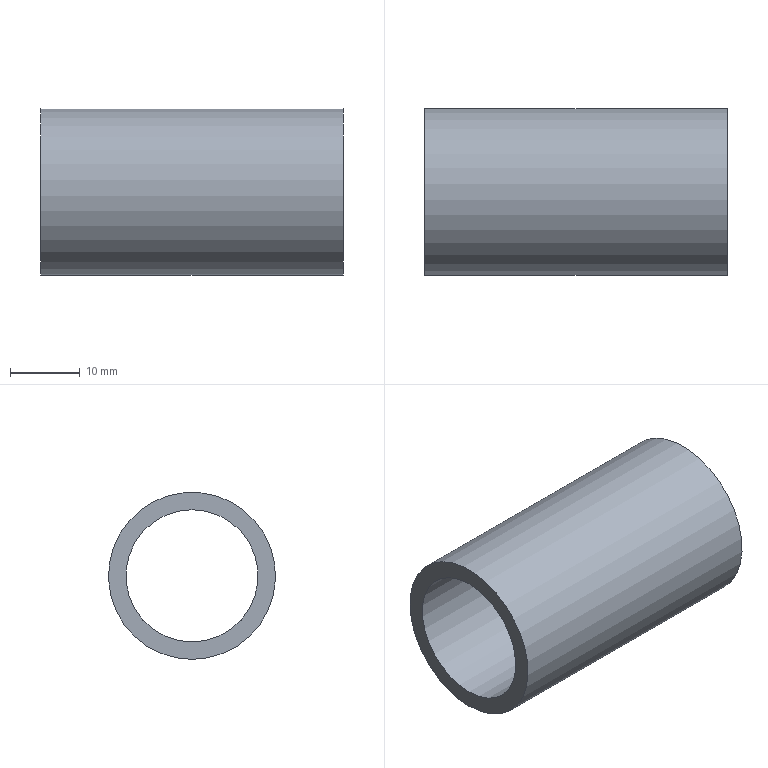Component | NX | LONG_BUSHING | 1 solid | 4 faces | box 43.5 x 24 x 24 mm | volume 7345 mm3 | cylinder 2 | plane 2 | commonest cylinder face diameters 24 x1 19 x1
STEP:
#1=CARTESIAN_POINT('',(0.,0.,0.));
#2=DIRECTION('',(0.,0.,1.));
#3=DIRECTION('',(1.,0.,0.));
#4=AXIS2_PLACEMENT_3D('',#1,#2,#3);
#5=CARTESIAN_POINT('',(-19.,0.,111.));
#6=VERTEX_POINT('',#5);
#7=CARTESIAN_POINT('',(-19.,0.,123.));
#8=DIRECTION('',(-1.,0.,0.));
#9=DIRECTION('',(0.,0.,-1.));
#10=AXIS2_PLACEMENT_3D('',#7,#8,#9);
#11=CIRCLE('',#10,12.);
#12=CARTESIAN_POINT('',(-19.,0.,123.));
#13=DIRECTION('',(-1.,0.,0.));
#14=DIRECTION('',(0.,0.,1.));
#15=AXIS2_PLACEMENT_3D('',#12,#13,#14);
#16=CYLINDRICAL_SURFACE('',#15,12.);
#17=CARTESIAN_POINT('',(3.142,0.));
#18=DIRECTION('',(1.,0.));
#19=VECTOR('',#18,1.);
#20=LINE('',#17,#19);
#21=(GEOMETRIC_REPRESENTATION_CONTEXT(2)PARAMETRIC_REPRESENTATION_CONTEXT()REPRESENTATION_CONTEXT('',''));
#22=DEFINITIONAL_REPRESENTATION('',(#20),#21);
#23=PCURVE('',#16,#22);
#24=CARTESIAN_POINT('',(-19.,0.,123.));
#25=DIRECTION('',(-1.,0.,0.));
#26=DIRECTION('',(0.,0.,1.));
#27=AXIS2_PLACEMENT_3D('',#24,#25,#26);
#28=PLANE('',#27);
#29=CARTESIAN_POINT('',(0.,0.));
#30=DIRECTION('',(-1.,0.));
#31=AXIS2_PLACEMENT_2D('',#29,#30);
#32=CIRCLE('',#31,12.);
#33=(GEOMETRIC_REPRESENTATION_CONTEXT(2)PARAMETRIC_REPRESENTATION_CONTEXT()REPRESENTATION_CONTEXT('',''));
#34=DEFINITIONAL_REPRESENTATION('',(#32),#33);
#35=PCURVE('',#28,#34);
#36=SURFACE_CURVE('',#11,(#23,#35),.PCURVE_S1.);
#37=EDGE_CURVE('',#6,#6,#36,.T.);
#38=ORIENTED_EDGE('',*,*,#37,.T.);
#39=CARTESIAN_POINT('',(-62.5,0.,111.));
#40=VERTEX_POINT('',#39);
#41=CARTESIAN_POINT('',(-19.,0.,111.));
#42=CARTESIAN_POINT('',(-62.5,0.,111.));
#43=B_SPLINE_CURVE_WITH_KNOTS('',1,(#41,#42),.UNSPECIFIED.,.F.,.F.,(2,2),(0.,43.5),.PIECEWISE_BEZIER_KNOTS.);
#44=CARTESIAN_POINT('',(9.425,0.));
#45=DIRECTION('',(0.,1.));
#46=VECTOR('',#45,1.);
#47=LINE('',#44,#46);
#48=(GEOMETRIC_REPRESENTATION_CONTEXT(2)PARAMETRIC_REPRESENTATION_CONTEXT()REPRESENTATION_CONTEXT('',''));
#49=DEFINITIONAL_REPRESENTATION('',(#47),#48);
#50=PCURVE('',#16,#49);
#51=CARTESIAN_POINT('',(3.142,0.));
#52=DIRECTION('',(0.,1.));
#53=VECTOR('',#52,1.);
#54=LINE('',#51,#53);
#55=(GEOMETRIC_REPRESENTATION_CONTEXT(2)PARAMETRIC_REPRESENTATION_CONTEXT()REPRESENTATION_CONTEXT('',''));
#56=DEFINITIONAL_REPRESENTATION('',(#54),#55);
#57=PCURVE('',#16,#56);
#58=SEAM_CURVE('',#43,(#50,#57),.PCURVE_S1.);
#59=EDGE_CURVE('',#6,#40,#58,.T.);
#60=ORIENTED_EDGE('',*,*,#59,.T.);
#61=CARTESIAN_POINT('',(-62.5,0.,123.));
#62=DIRECTION('',(-1.,0.,0.));
#63=DIRECTION('',(0.,0.,-1.));
#64=AXIS2_PLACEMENT_3D('',#61,#62,#63);
#65=CIRCLE('',#64,12.);
#66=CARTESIAN_POINT('',(3.142,43.5));
#67=DIRECTION('',(1.,0.));
#68=VECTOR('',#67,1.);
#69=LINE('',#66,#68);
#70=(GEOMETRIC_REPRESENTATION_CONTEXT(2)PARAMETRIC_REPRESENTATION_CONTEXT()REPRESENTATION_CONTEXT('',''));
#71=DEFINITIONAL_REPRESENTATION('',(#69),#70);
#72=PCURVE('',#16,#71);
#73=CARTESIAN_POINT('',(-62.5,0.,123.));
#74=DIRECTION('',(-1.,0.,0.));
#75=DIRECTION('',(0.,0.,1.));
#76=AXIS2_PLACEMENT_3D('',#73,#74,#75);
#77=PLANE('',#76);
#78=CARTESIAN_POINT('',(0.,0.));
#79=DIRECTION('',(-1.,0.));
#80=AXIS2_PLACEMENT_2D('',#78,#79);
#81=CIRCLE('',#80,12.);
#82=(GEOMETRIC_REPRESENTATION_CONTEXT(2)PARAMETRIC_REPRESENTATION_CONTEXT()REPRESENTATION_CONTEXT('',''));
#83=DEFINITIONAL_REPRESENTATION('',(#81),#82);
#84=PCURVE('',#77,#83);
#85=SURFACE_CURVE('',#65,(#72,#84),.PCURVE_S1.);
#86=EDGE_CURVE('',#40,#40,#85,.T.);
#87=ORIENTED_EDGE('',*,*,#86,.F.);
#88=ORIENTED_EDGE('',*,*,#59,.F.);
#89=EDGE_LOOP('',(#38,#60,#87,#88));
#90=FACE_BOUND('',#89,.T.);
#91=ADVANCED_FACE('',(#90),#16,.T.);
#92=CARTESIAN_POINT('',(-19.,0.,113.5));
#93=VERTEX_POINT('',#92);
#94=CARTESIAN_POINT('',(-19.,0.,123.));
#95=DIRECTION('',(-1.,0.,0.));
#96=DIRECTION('',(0.,0.,-1.));
#97=AXIS2_PLACEMENT_3D('',#94,#95,#96);
#98=CIRCLE('',#97,9.5);
#99=CARTESIAN_POINT('',(-19.,0.,123.));
#100=DIRECTION('',(-1.,0.,0.));
#101=DIRECTION('',(0.,0.,1.));
#102=AXIS2_PLACEMENT_3D('',#99,#100,#101);
#103=CYLINDRICAL_SURFACE('',#102,9.5);
#104=CARTESIAN_POINT('',(3.142,0.));
#105=DIRECTION('',(1.,0.));
#106=VECTOR('',#105,1.);
#107=LINE('',#104,#106);
#108=(GEOMETRIC_REPRESENTATION_CONTEXT(2)PARAMETRIC_REPRESENTATION_CONTEXT()REPRESENTATION_CONTEXT('',''));
#109=DEFINITIONAL_REPRESENTATION('',(#107),#108);
#110=PCURVE('',#103,#109);
#111=CARTESIAN_POINT('',(0.,0.));
#112=DIRECTION('',(-1.,0.));
#113=AXIS2_PLACEMENT_2D('',#111,#112);
#114=CIRCLE('',#113,9.5);
#115=(GEOMETRIC_REPRESENTATION_CONTEXT(2)PARAMETRIC_REPRESENTATION_CONTEXT()REPRESENTATION_CONTEXT('',''));
#116=DEFINITIONAL_REPRESENTATION('',(#114),#115);
#117=PCURVE('',#28,#116);
#118=SURFACE_CURVE('',#98,(#110,#117),.PCURVE_S1.);
#119=EDGE_CURVE('',#93,#93,#118,.T.);
#120=ORIENTED_EDGE('',*,*,#119,.T.);
#121=CARTESIAN_POINT('',(-62.5,0.,113.5));
#122=VERTEX_POINT('',#121);
#123=CARTESIAN_POINT('',(-19.,0.,113.5));
#124=CARTESIAN_POINT('',(-62.5,0.,113.5));
#125=B_SPLINE_CURVE_WITH_KNOTS('',1,(#123,#124),.UNSPECIFIED.,.F.,.F.,(2,2),(0.,43.5),.PIECEWISE_BEZIER_KNOTS.);
#126=CARTESIAN_POINT('',(9.425,0.));
#127=DIRECTION('',(0.,1.));
#128=VECTOR('',#127,1.);
#129=LINE('',#126,#128);
#130=(GEOMETRIC_REPRESENTATION_CONTEXT(2)PARAMETRIC_REPRESENTATION_CONTEXT()REPRESENTATION_CONTEXT('',''));
#131=DEFINITIONAL_REPRESENTATION('',(#129),#130);
#132=PCURVE('',#103,#131);
#133=CARTESIAN_POINT('',(3.142,0.));
#134=DIRECTION('',(0.,1.));
#135=VECTOR('',#134,1.);
#136=LINE('',#133,#135);
#137=(GEOMETRIC_REPRESENTATION_CONTEXT(2)PARAMETRIC_REPRESENTATION_CONTEXT()REPRESENTATION_CONTEXT('',''));
#138=DEFINITIONAL_REPRESENTATION('',(#136),#137);
#139=PCURVE('',#103,#138);
#140=SEAM_CURVE('',#125,(#132,#139),.PCURVE_S1.);
#141=EDGE_CURVE('',#93,#122,#140,.T.);
#142=ORIENTED_EDGE('',*,*,#141,.T.);
#143=CARTESIAN_POINT('',(-62.5,0.,123.));
#144=DIRECTION('',(-1.,0.,0.));
#145=DIRECTION('',(0.,0.,-1.));
#146=AXIS2_PLACEMENT_3D('',#143,#144,#145);
#147=CIRCLE('',#146,9.5);
#148=CARTESIAN_POINT('',(3.142,43.5));
#149=DIRECTION('',(1.,0.));
#150=VECTOR('',#149,1.);
#151=LINE('',#148,#150);
#152=(GEOMETRIC_REPRESENTATION_CONTEXT(2)PARAMETRIC_REPRESENTATION_CONTEXT()REPRESENTATION_CONTEXT('',''));
#153=DEFINITIONAL_REPRESENTATION('',(#151),#152);
#154=PCURVE('',#103,#153);
#155=CARTESIAN_POINT('',(0.,0.));
#156=DIRECTION('',(-1.,0.));
#157=AXIS2_PLACEMENT_2D('',#155,#156);
#158=CIRCLE('',#157,9.5);
#159=(GEOMETRIC_REPRESENTATION_CONTEXT(2)PARAMETRIC_REPRESENTATION_CONTEXT()REPRESENTATION_CONTEXT('',''));
#160=DEFINITIONAL_REPRESENTATION('',(#158),#159);
#161=PCURVE('',#77,#160);
#162=SURFACE_CURVE('',#147,(#154,#161),.PCURVE_S1.);
#163=EDGE_CURVE('',#122,#122,#162,.T.);
#164=ORIENTED_EDGE('',*,*,#163,.F.);
#165=ORIENTED_EDGE('',*,*,#141,.F.);
#166=EDGE_LOOP('',(#120,#142,#164,#165));
#167=FACE_BOUND('',#166,.F.);
#168=ADVANCED_FACE('',(#167),#103,.F.);
#169=ORIENTED_EDGE('',*,*,#37,.F.);
#170=EDGE_LOOP('',(#169));
#171=FACE_BOUND('',#170,.T.);
#172=ORIENTED_EDGE('',*,*,#119,.T.);
#173=EDGE_LOOP('',(#172));
#174=FACE_BOUND('',#173,.T.);
#175=ADVANCED_FACE('',(#171,#174),#28,.F.);
#176=ORIENTED_EDGE('',*,*,#86,.T.);
#177=EDGE_LOOP('',(#176));
#178=FACE_BOUND('',#177,.T.);
#179=ORIENTED_EDGE('',*,*,#163,.F.);
#180=EDGE_LOOP('',(#179));
#181=FACE_BOUND('',#180,.T.);
#182=ADVANCED_FACE('',(#178,#181),#77,.T.);
#183=CLOSED_SHELL('',(#91,#168,#175,#182));
#184=MANIFOLD_SOLID_BREP('',#183);
#185=(LENGTH_UNIT()NAMED_UNIT(*)SI_UNIT(.MILLI.,.METRE.));
#186=UNCERTAINTY_MEASURE_WITH_UNIT(LENGTH_MEASURE(0.00001),#185,'','');
#187=(NAMED_UNIT(*)PLANE_ANGLE_UNIT()SI_UNIT($,.RADIAN.));
#188=(NAMED_UNIT(*)SI_UNIT($,.STERADIAN.)SOLID_ANGLE_UNIT());
#189=(GEOMETRIC_REPRESENTATION_CONTEXT(3)GLOBAL_UNCERTAINTY_ASSIGNED_CONTEXT((#186))GLOBAL_UNIT_ASSIGNED_CONTEXT((#185,#187,#188))REPRESENTATION_CONTEXT('',''));
#190=ADVANCED_BREP_SHAPE_REPRESENTATION('',(#4,#184),#189);